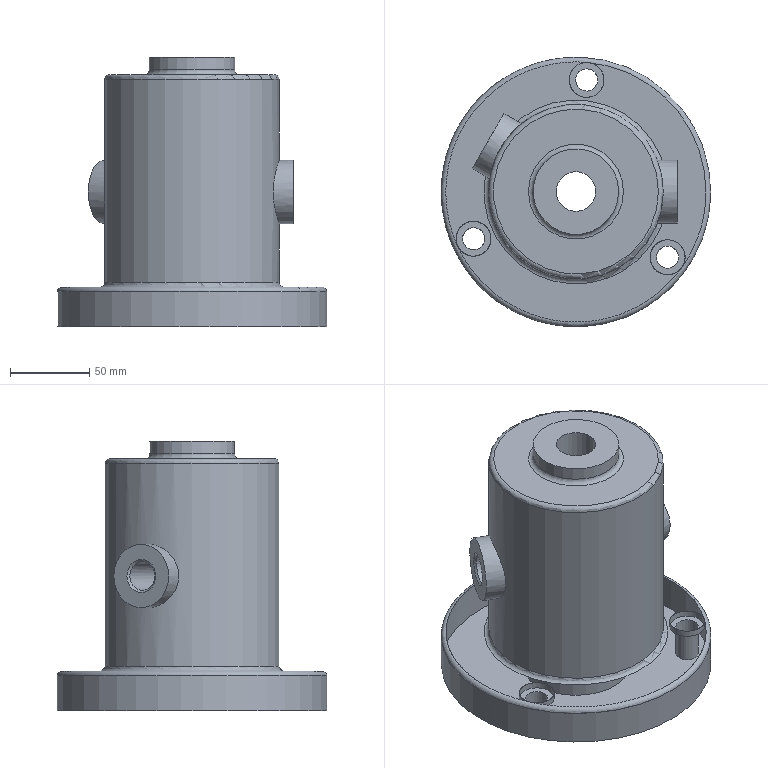CAM job | NX | mm | 3-axis | 1 set-up | 1 operations | part box 170 x 170 x 170
set-up 1
1. Cavity Milling | Mill Mill5 MILLD10 | CAVITY_MILL | path 732314.023 mm | 1327.165 min